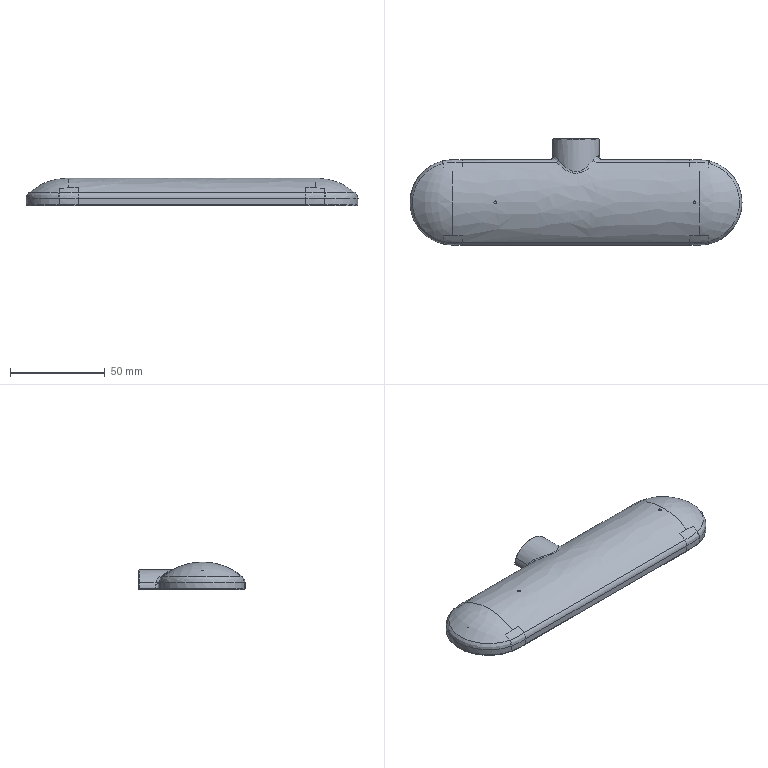Component | NX | SHANGDENGKE | 1 solid | 151 faces | volume 11170 mm3 | spline 70 | plane 37 | cylinder 32 | torus 7 | cone 5 | commonest cylinder face diameters 1.5 x7 5 x5 8 x3 6 x3 24 x2 43 x2 45 x2 11.25 x2